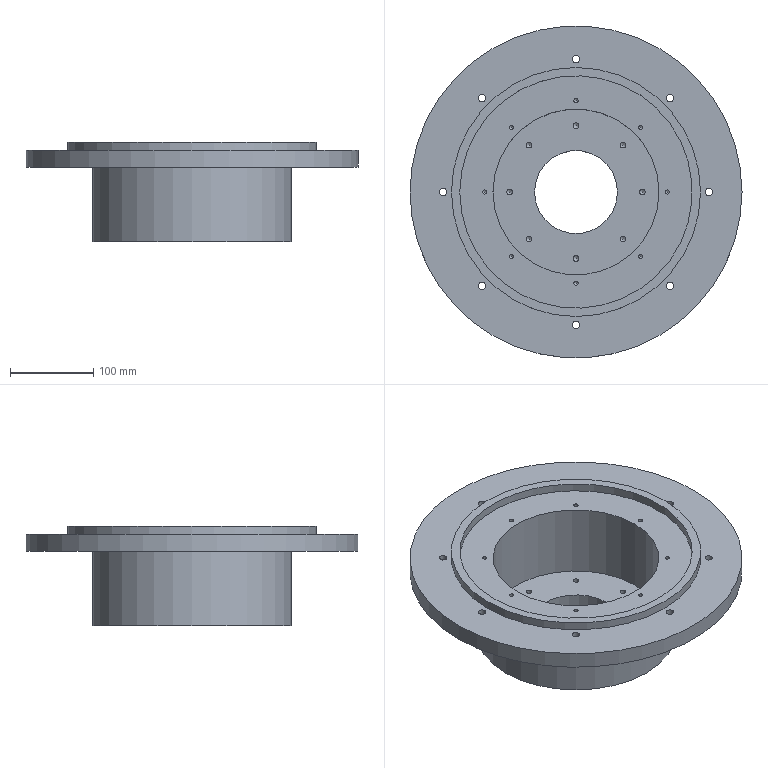Component | NX | BALL_BASE | 1 solid | 68 faces | volume 3666421 mm3 | cylinder 38 | cone 16 | plane 14 | commonest cylinder face diameters 9 x8 15 x8 5 x8 6.8 x8 400 x1 240 x1 100 x1 200 x1